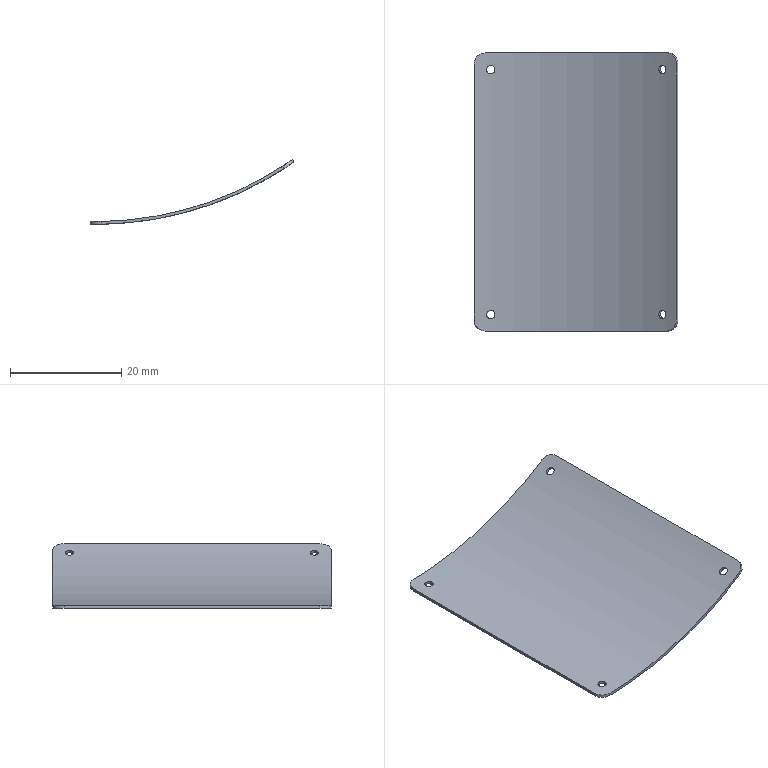Component | SolidWorks | Plaque signal_tique Festo-1 | 1 solid | 756 faces | box 36.63 x 50 x 11.62 mm | volume 889 mm3 | plane 397 | spline 330 | cylinder 29 | commonest cylinder face diameters 124.98 x11 1.5 x8 4 x4 2 x4 125 x1 124 x1